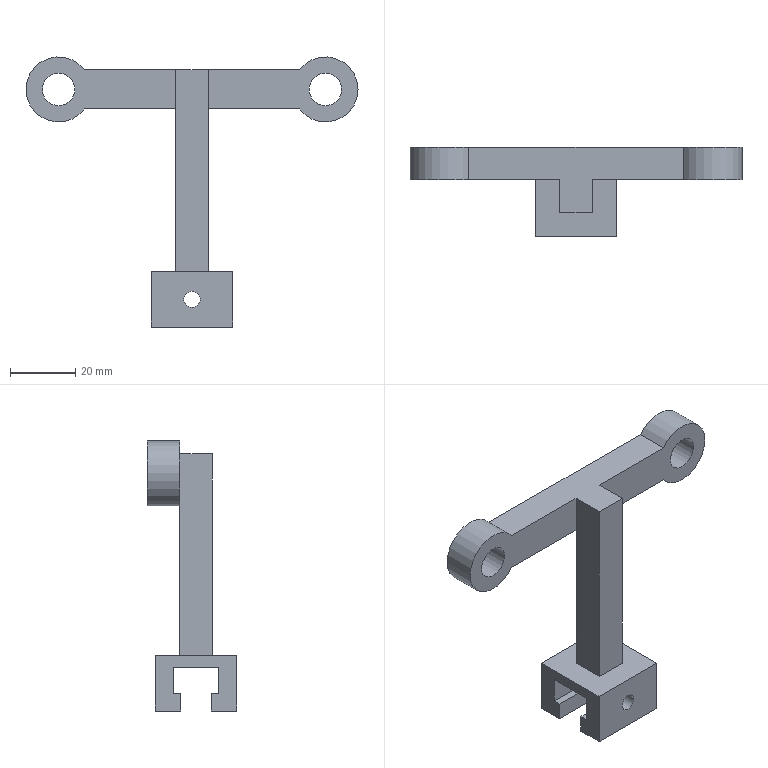Component | NX | CONNECTING_ROD_BRACKET | 1 solid | 29 faces | volume 24831 mm3 | plane 23 | cylinder 6 | commonest cylinder face diameters 20 x2 10 x2 5 x2